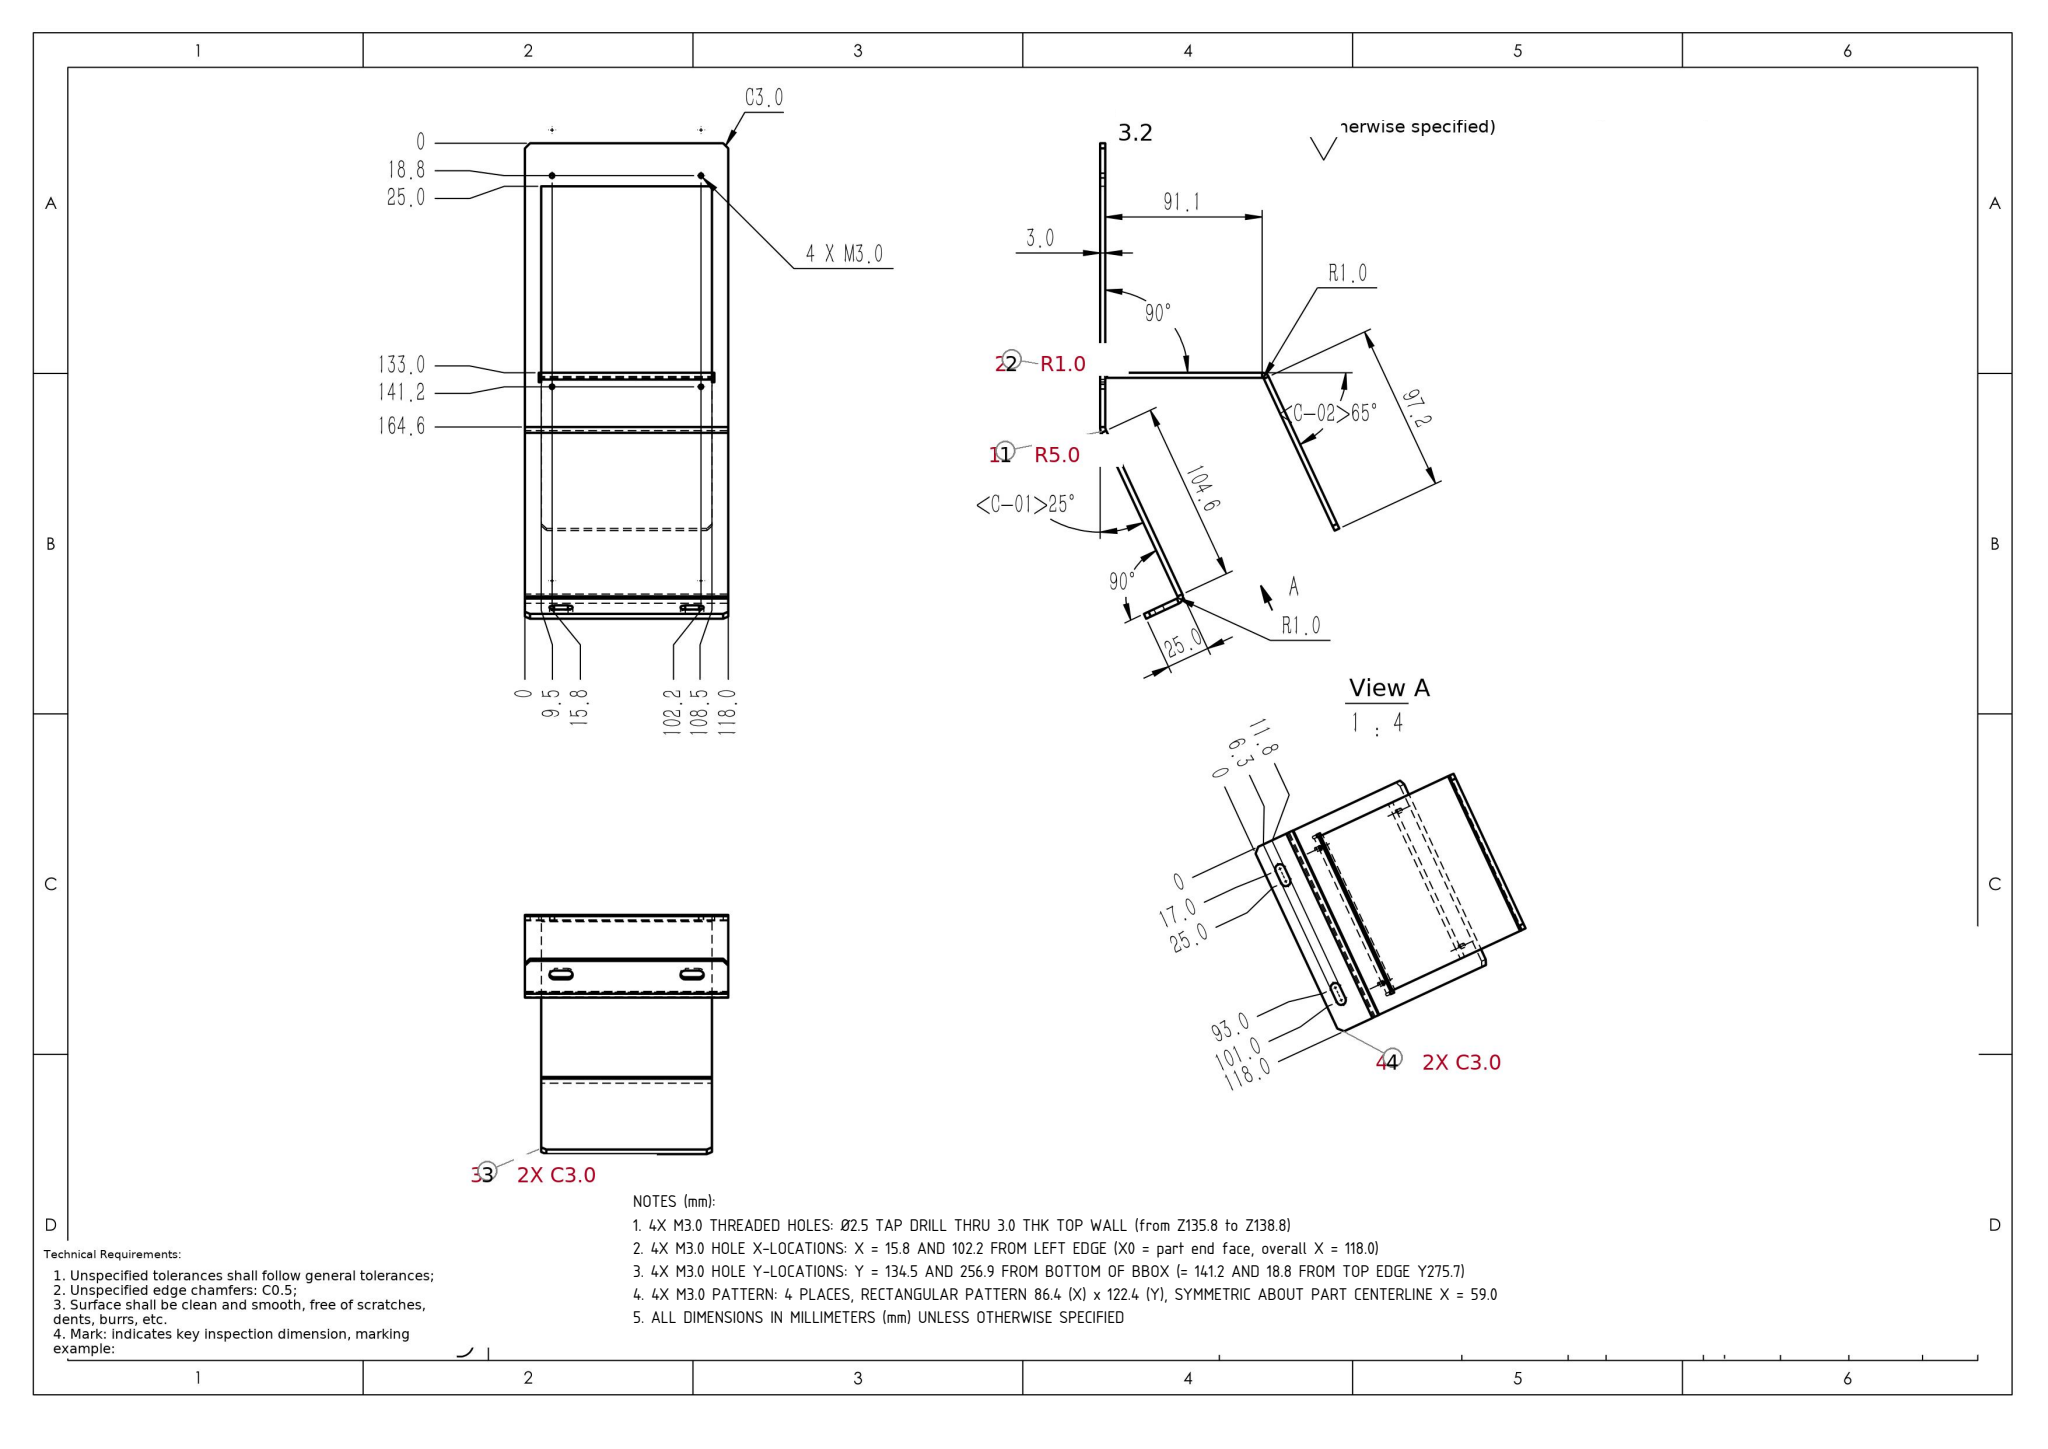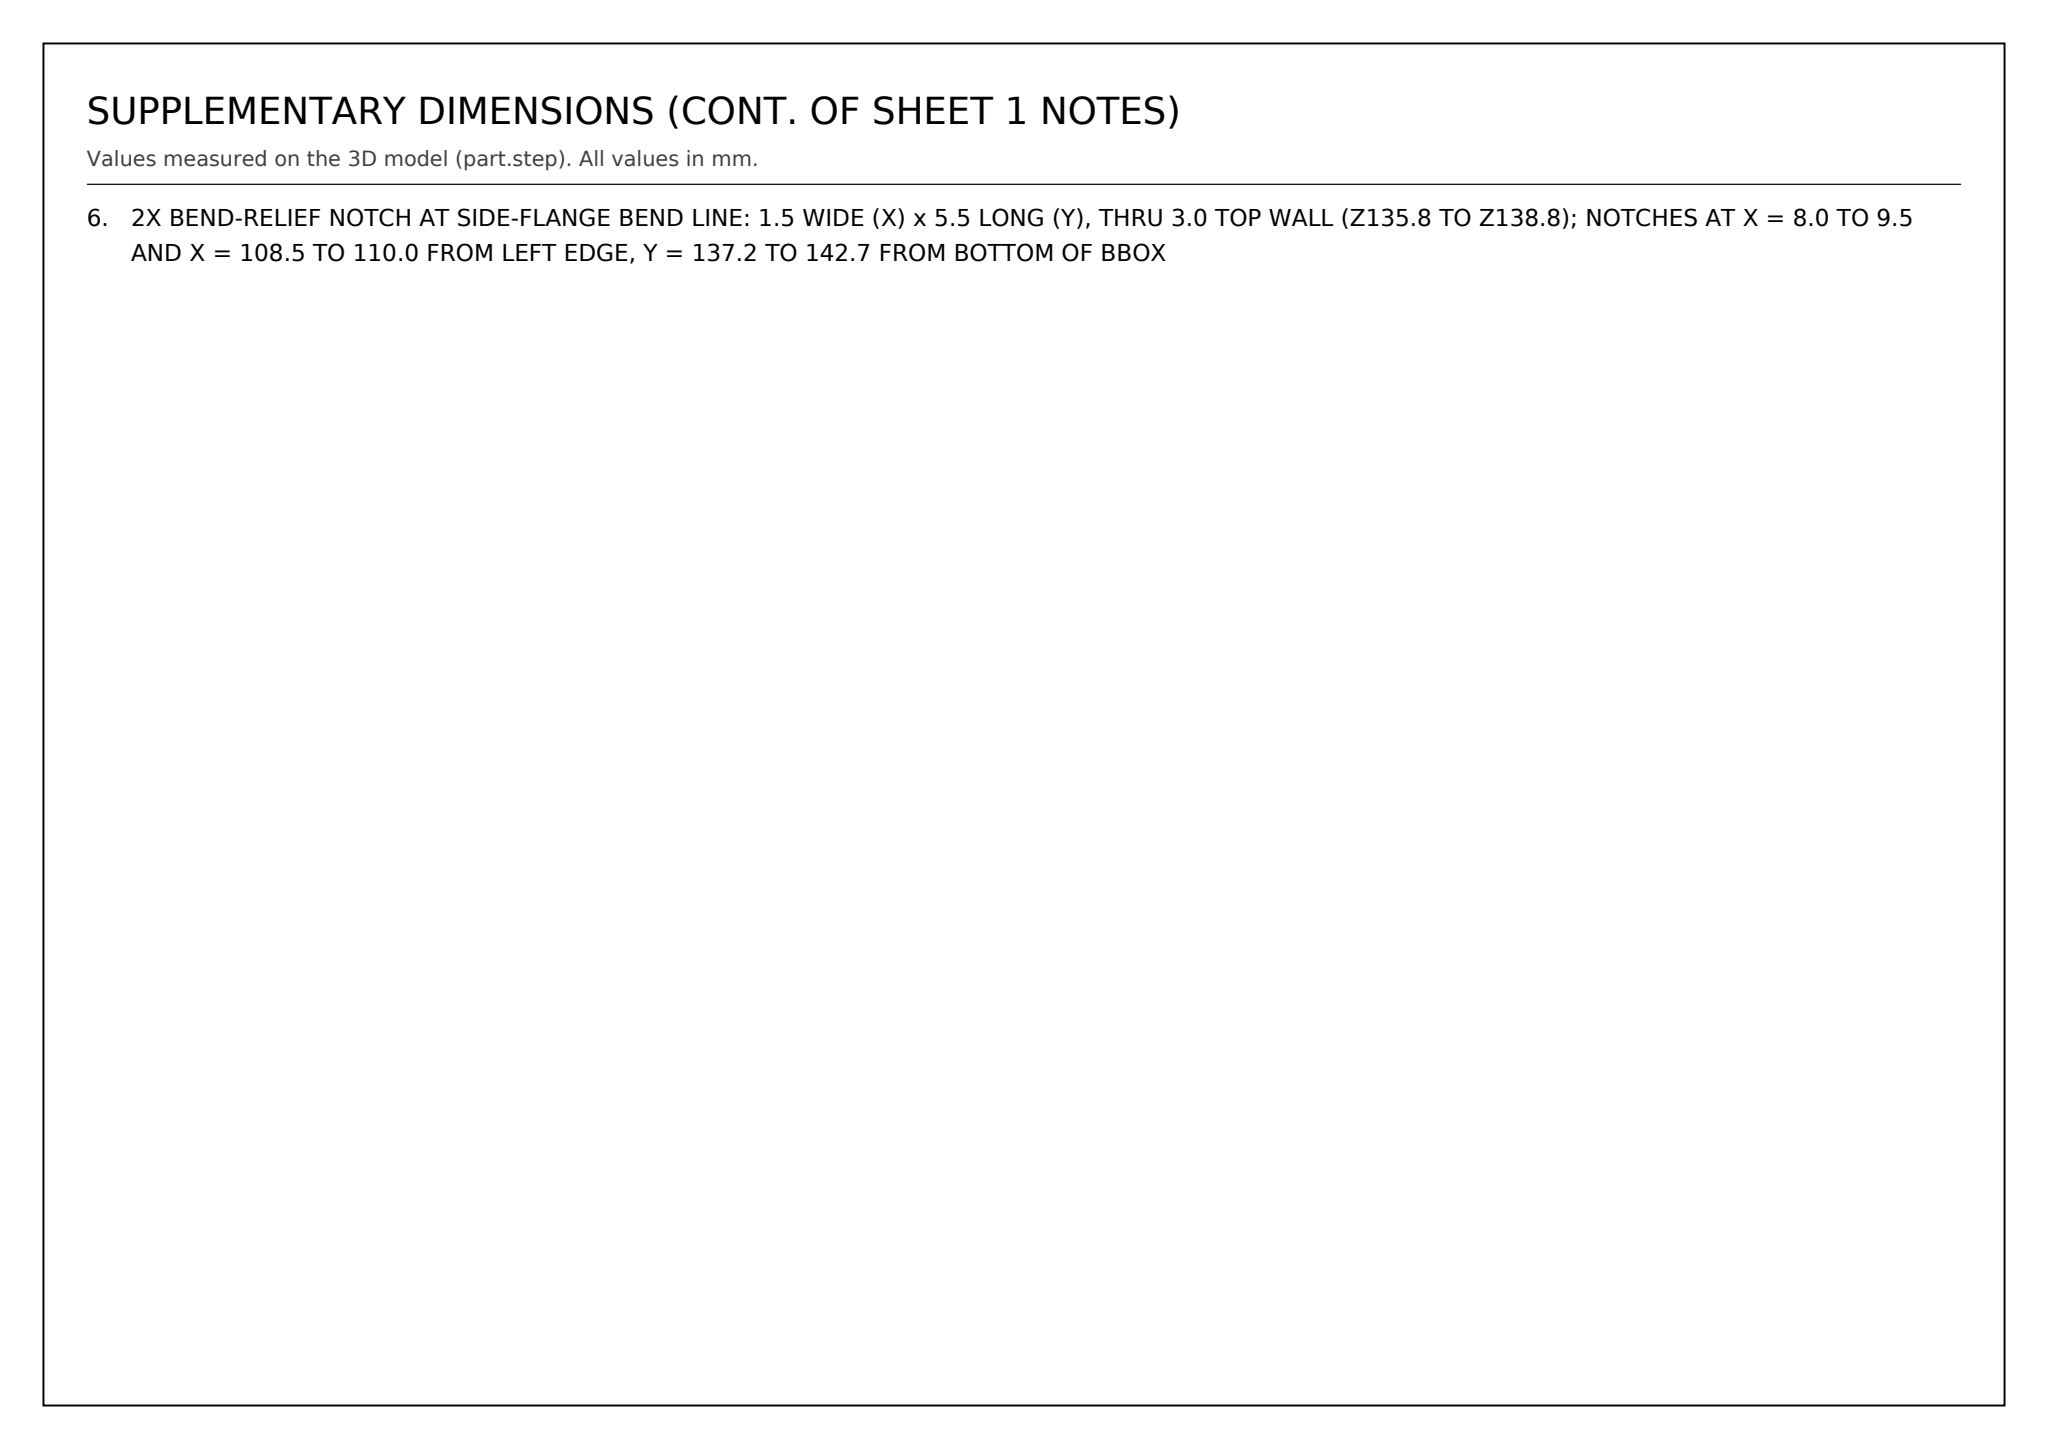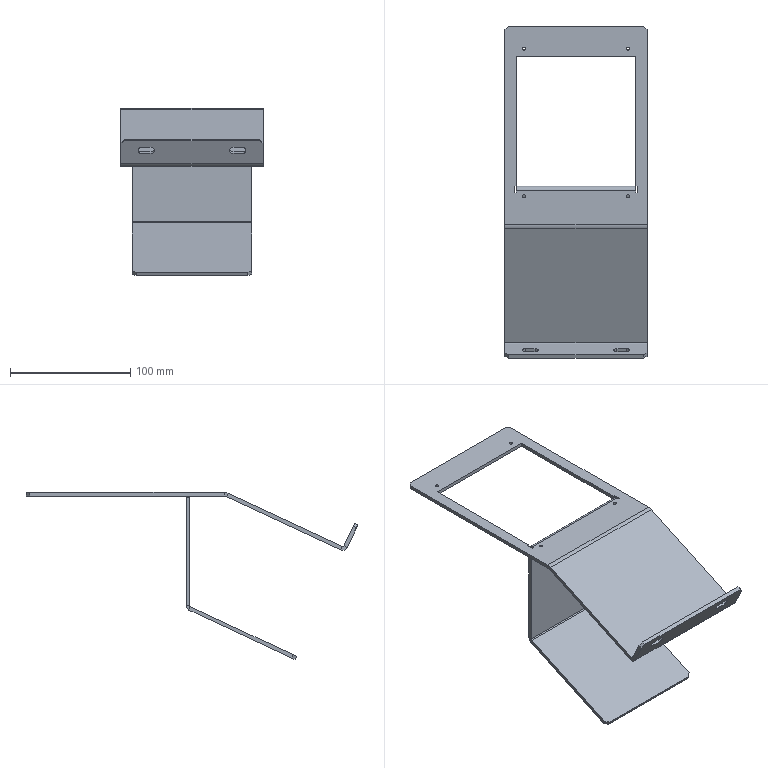Part | SolidWorks | mm | 1 solid | 72 faces | box 118 x 275.67 x 138.77 mm | volume 128881 mm3 | plane 52 | cylinder 20 | commonest cylinder face diameters 2.5 x8 5.5 x4 8 x3 2 x3 10 x1 16 x1
Drawing notes:
4X M3.0 THREADED HOLES: Ø2.5 TAP DRILL THRU 3.0 THK TOP WALL (from Z135.8 to Z138.8) | from the solid: cylinders: 4X 'hole/bore' dia 2.5, axis z, from 135.8 to 138.8 (wall thickness 3.0 = plane z135.8 to z138.8)
4X M3.0 HOLE X-LOCATIONS: X = 15.8 AND 102.2 FROM LEFT EDGE (X0 = part end face, overall X = 118.0) | from the solid: cylinders: holes dia 2.5 at x = 15.8 and 102.2; axis_planes x = 0.0 and x = 118.0 (bbox_xyz X = 118.0)
4X M3.0 HOLE Y-LOCATIONS: Y = 134.5 AND 256.9 FROM BOTTOM OF BBOX (= 141.2 AND 18.8 FROM TOP EDGE Y275.7) | from the solid: cylinders: holes dia 2.5 at y = 134.5 and 256.9; axis_plane y = 275.7 (top edge)
4X M3.0 PATTERN: 4 PLACES, RECTANGULAR PATTERN 86.4 (X) x 122.4 (Y), SYMMETRIC ABOUT PART CENTERLINE X = 59.0 | from the solid: cylinders: hole dia 2.5 at (15.8/102.2, 134.5/256.9) -> spacing 102.2-15.8 = 86.4 and 256.9-134.5 = 122.4; bbox X 118.0 gives centerline 59.0
ALL DIMENSIONS IN MILLIMETERS (mm) UNLESS OTHERWISE SPECIFIED | from the solid: STEP model facts header: units mm; bbox_xyz [118.0, 275.669, 138.766]
2X BEND-RELIEF NOTCH AT SIDE-FLANGE BEND LINE: 1.5 WIDE (X) x 5.5 LONG (Y), THRU 3.0 TOP WALL (Z135.8 TO Z138.8); NOTCHES AT X = 8.0 TO 9.5 AND X = 108.5 TO 110.0 FROM LEFT EDGE, Y = 137.2 TO 142.7 FROM BOTTOM OF BBOX | from the solid: axis_planes x=8.0 extent y[137.2,142.7] z[135.8,138.8] and x=110.0 extent y[137.2,142.7] z[135.8,138.8]; end faces x=9.5 and x=108.5 extent y[137.2,138.7] z[135.8,138.8]; y=137.2 planes x[8.0,9.5] and x[108.5,110.0] z[135.8,138.8]